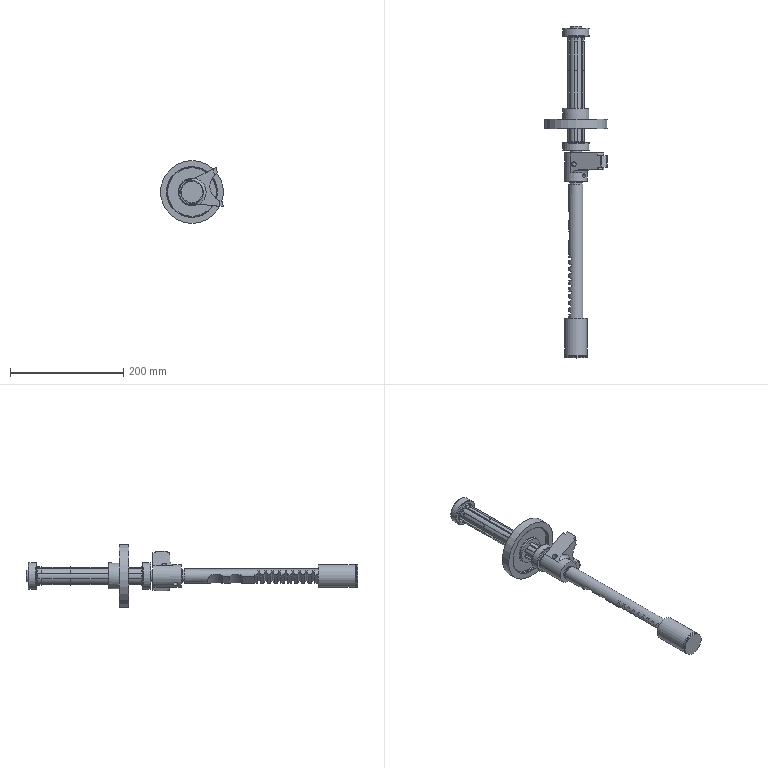Assembly | NX | mm | 7 component files | 9 solids | 260 faces | box 111 x 586 x 111 mm | volume 568969 mm3 | plane 149 | cylinder 86 | torus 17 | cone 8 | commonest cylinder face diameters 32 x24 26 x12 30 x12 20 x5 30.5 x4 36.5 x4 40 x3 8 x3
Bill of materials:
unnamed part 1 | 1 |  | Flanged hub: a wide thin circular flange with a smaller coaxial cylindrical boss on one side, and a central through bore with six evenly spaced rectangular internal notches (a spline-like or keyed bore).
unnamed part 2 | 1 |  | Long slender cylindrical rod with a short reduced-diameter stepped end that has a transverse cross hole, and a row of evenly spaced rectangular notches cut along one side over part of its length (rack-like teeth).
unnamed part 3 | 2 |  | Annular ring assembly-like body: a concentric outer ring and inner ring of equal width separated by an open annular gap, with rounded edges and a central through bore; it looks like a simplified bearing.
unnamed part 4 | 1 |  | Solid plain cylinder (pin or short shaft) with flat ends and a narrow circumferential groove near one end.
unnamed part 5 | 1 |  | Splined shaft: a central cylindrical section carrying six evenly spaced longitudinal rectangular ribs/splines, with smaller-diameter plain cylindrical journals at both ends.
unnamed part 6 | 1 |  | Bracket/housing: a cylindrical boss with a stepped through bore merging into a flared plate-like body that ends in a wide fork with a large concave arc cutout and stepped notches/slots on its arms.
Mates:
1. touch align | model3 1 | model1 1
2. touch align | model5 1 | model1 1
3. touch align | model3 1 | model1 1
4. touch align | zhou9 1 face | zhou9-chulun2 1 face
5. touch align | zhou9 1 face | zhou9-chulun2 1 face
6. touch align | zhou9 1 face | zhou9-chulun2 1 face
7. touch align | zhou9 1 face | gundongzhoucheng9 2 face
8. touch align | zhou9 1 face | gundongzhoucheng9 2 face
9. touch align | zhou9 1 face | gundongzhoucheng9 1 face